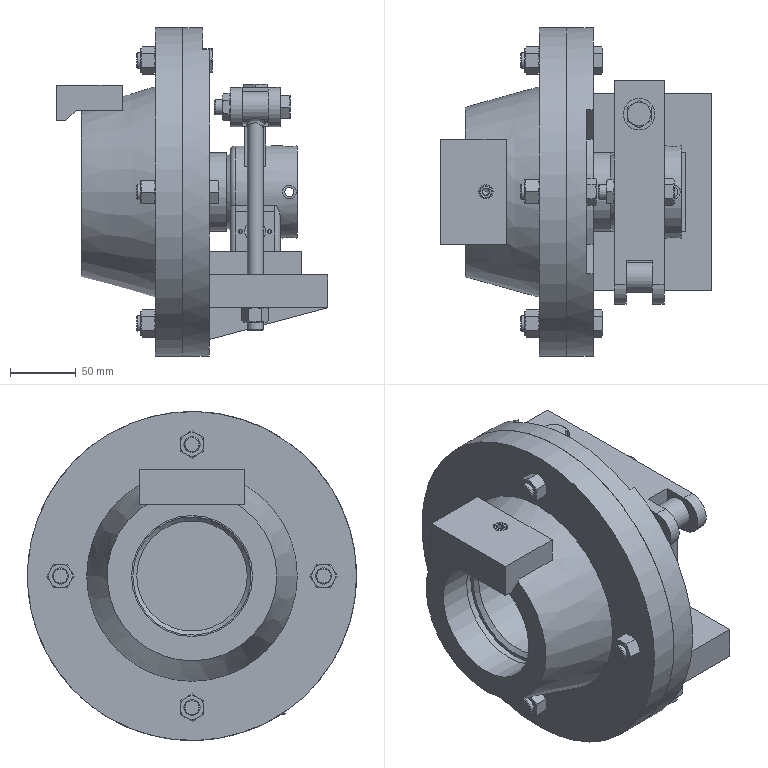Assembly | NX | mm | 28 component files | 28 solids | 606 faces | box 206 x 250 x 250 mm | volume 3239460 mm3 | plane 284 | cone 190 | cylinder 109 | torus 20 | spline 3 | commonest cylinder face diameters 12 x15 13 x8 3.3 x8 11.701 x6 10 x6 4 x6 6 x5 2.874 x4
Bill of materials:
unnamed part 1 | 1 |  | Rectangular block with one offset vertical hole and a stepped, angled underside on one end.
unnamed part 2 | 1 |  | Hollow cylindrical housing with an annular end face drilled with four holes, radial side holes, and a rectangular block extension that carries a bore and a small hole/slot pattern.
unnamed part 3 | 1 |  | Flanged hub: a circular flange with four through holes and a tapered conical boss on one side, with a stepped central bore.
GB-T5780-2000,M12x55 | 3 |  | Hex-head bolt-like part: a straight plain cylindrical shank with a hexagonal prism head at one end. The head has chamfered corners that form a circular face on its outer end.
GB-T70.1-2000,M3x8 | 4 |  | Hexagon Socket Head Cap Screw, GB-T 70.1-2000,M3x8
unnamed part 4 | 1 |  | Flat annular ring with a large central opening and four equally spaced axial through holes.
GB-T6172_1-2000,M12x1.75 | 1 |  | Hexagon Thin Nut, Chamfered, GB-T 6172.1-2000,M12x1.75
GB-T119.1-2000,10x35 | 1 |  | Parallel Pin, GB-T 119.1-2000,10x35
GB-T5780-2000,M12x50 | 2 |  | Hex-head bolt-like part: a straight plain cylindrical shank with a hexagonal prism head at one end. The head has chamfered corners that form a circular face on its outer end. It is almost the same as the other part, but its shank looks slightly thicker compared with its length and the head.
GB-T6170_F-2000,M12x1.75 | 6 |  | Hexagonal nut shape with chamfered corners and a plain round central bore.
unnamed part 5 | 1 |  | Long slender cylindrical rod with a cylindrical eye at one end; the eye has a through hole perpendicular to the rod axis.
unnamed part 6 | 1 |  | Bolt-like part: a hexagonal head on a long plain cylindrical shank.
unnamed part 7 | 1 |  | Rectangular bar with a clevis-style fork at one rounded end, a cross hole through the fork, a transverse side hole in the middle, and a counterbored vertical hole near the other end.
unnamed part 8 | 1 |  | Circular plate with a perpendicular rectangular tab on its lower face, plus an arc slot, through holes and small marks.
unnamed part 9 | 1 |  | Plain rectangular block or plate with no visible holes or features.
unnamed part 10 | 1 |  | Flat plate with an arc-shaped top edge, one through hole, and a V-shaped bottom notch ending in a small rectangular slot.
GB-T70.1-2000,M6x20 | 1 |  | Hexagon Socket Head Cap Screw, GB-T 70.1-2000,M6x20
Mates:
1. concentric | Adapter_plate 1 edge | Fixture_body 1 edge
2. touch align | Support_ring 1 face | Fixture_body 1 face
3. touch align | Support_ring 1 face | Fixture_body 1 face
4. touch align | Support_ring 1 face | Fixture_body 1 face
5. concentric | Gearbox 1 edge | Support_ring 1 edge
6. concentric | V_block 1 edge | Clamp_plate 1 edge
7. distance | V_block 1 point | assembly datumplane
8. touch align | V_block 1 face | Gearbox 1 face
9. parallel | Clamp_plate 1 face | Fixture_body 1 face
10. fix | Adapter_plate 1 component
11. perpendicular | V_block 1 face | Clamp_plate 1 face
12. touch align | Fixture_body 1 face | Adapter_plate 1 face
13. parallel | Gearbox 1 face | Fixture_body 1 face
14. distance | Clamp_plate 1 point | Fixture_body 1 face
15. concentric | Screw_M12 1 edge | Clamp_plate 1 edge
16. concentric | Bolt_M12x170 1 edge | Clamp_plate 1 edge
17. concentric | GB-T5780-2000_M12x50 2 edge | Clamp_plate 1 edge
18. concentric | GB-T6172_1-2000_M12x1_75 1 arc | Clamp_plate 1 edge
19. concentric | GB-T6170_F-2000_M12x1_75 6 edge | Fixture_body 1 edge
20. concentric | GB-T6170_F-2000_M12x1_75 5 edge | Fixture_body 1 edge
21. concentric | GB-T70_1-2000_M3x8 4 edge | Support_ring 1 edge
22. bond | Support_ring 1 component | assembly component
23. bond | GB-T70_1-2000_M3x8 4 component | assembly component
24. bond | GB-T70_1-2000_M3x8 3 component | assembly component
25. bond | GB-T70_1-2000_M3x8 2 component | assembly component
26. bond | GB-T70_1-2000_M3x8 1 component | assembly component
27. circular | assembly datumaxis | assembly cartesiancoordinatesystem | assembly cartesiancoordinatesystem | assembly cartesiancoordinatesystem | assembly cartesiancoordinatesystem
28. center | Support_plate 1 face | Support_plate 1 face | Fixture_body 1 face | Fixture_body 1 face
29. distance | Support_plate 1 face | Gearbox 1 face
30. touch align | Support_plate 1 face | Fixture_body 1 face
31. concentric | GB-T5780-2000_M12x55 3 edge | Fixture_body 1 edge
32. bond | Fixture_body 1 component | assembly component
33. bond | GB-T5780-2000_M12x55 3 component | assembly component
34. bond | GB-T5780-2000_M12x55 2 component | assembly component
35. bond | GB-T5780-2000_M12x55 1 component | assembly component
36. circular | assembly datumaxis | assembly cartesiancoordinatesystem | assembly cartesiancoordinatesystem | assembly cartesiancoordinatesystem
37. touch align | GB-T5780-2000_M12x50 1 face | Adapter_plate 1 face
38. touch align | GB-T5780-2000_M12x50 1 face | Fixture_body 1 face
39. concentric | GB-T6170_F-2000_M12x1_75 4 edge | Adapter_plate 1 edge
40. bond | Adapter_plate 1 component | assembly component
41. bond | GB-T6170_F-2000_M12x1_75 4 component | assembly component
42. bond | GB-T6170_F-2000_M12x1_75 3 component | assembly component
43. bond | GB-T6170_F-2000_M12x1_75 2 component | assembly component
44. circular | assembly datumaxis | assembly cartesiancoordinatesystem | assembly cartesiancoordinatesystem | assembly cartesiancoordinatesystem | assembly cartesiancoordinatesystem
45. bond | GB-T6170_F-2000_M12x1_75 1 component | assembly component
46. concentric | 1 1 edge | Adapter_plate 1 arc
47. concentric | GB-T70_1-2000_M6x20 1 edge | 1 1 edge
48. concentric | GB-T119_1-2000_10x35 1 edge | Clamp_plate 1 edge